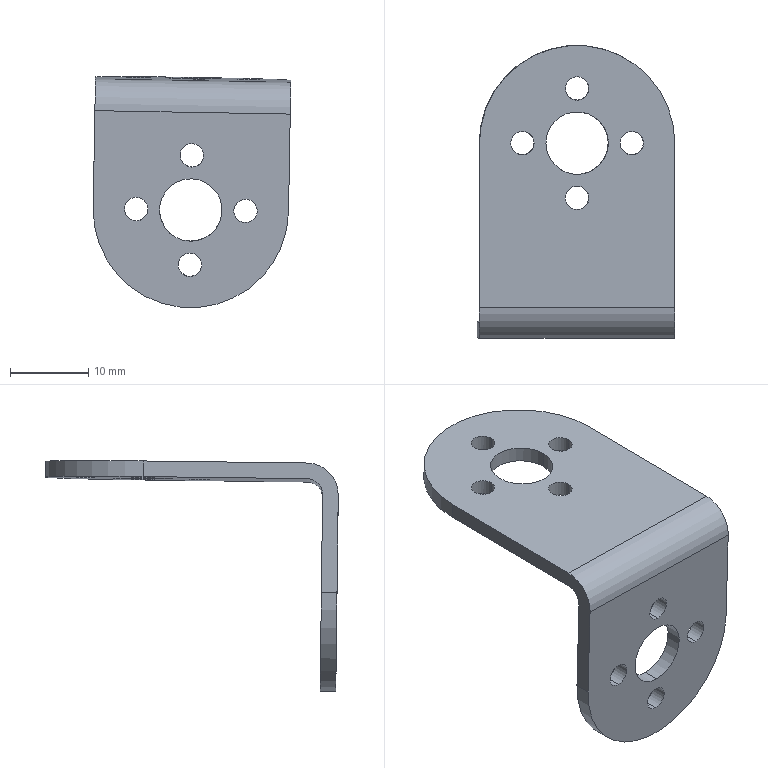Component | SolidWorks | L Shape Bracket-1 | 1 solid | 30 faces | box 25.29 x 37.47 x 29.58 mm | volume 2578 mm3 | cylinder 24 | plane 6 | commonest cylinder face diameters 3 x16 8 x5 25 x2 4 x1
STEP:
#1=COLOUR_RGB('',0.7922,0.8196,0.9333);
#2=FILL_AREA_STYLE_COLOUR('',#1);
#3=FILL_AREA_STYLE('',(#2));
#4=SURFACE_STYLE_FILL_AREA(#3);
#5=SURFACE_SIDE_STYLE('',(#4));
#6=SURFACE_STYLE_USAGE(.BOTH.,#5);
#7=PRESENTATION_STYLE_ASSIGNMENT((#6));
#8=CARTESIAN_POINT('',(1.258,4.504,1.069));
#9=VERTEX_POINT('',#8);
#10=CARTESIAN_POINT('',(1.261,4.659,1.228));
#11=VERTEX_POINT('',#10);
#12=CARTESIAN_POINT('',(1.258,4.661,1.071));
#13=DIRECTION('',(-0.9998,0.,0.01745));
#14=DIRECTION('',(0.01218,-0.716,0.698));
#15=AXIS2_PLACEMENT_3D('',#12,#13,#14);
#16=CIRCLE('',#15,0.1575);
#17=EDGE_CURVE('',#9,#11,#16,.T.);
#18=ORIENTED_EDGE('',*,*,#17,.T.);
#19=CARTESIAN_POINT('',(0.2769,4.659,1.246));
#20=VERTEX_POINT('',#19);
#21=CARTESIAN_POINT('',(0.5229,4.659,1.241));
#22=DIRECTION('',(-0.9998,0.,0.01745));
#23=VECTOR('',#22,39.37);
#24=LINE('',#21,#23);
#25=EDGE_CURVE('',#11,#20,#24,.T.);
#26=ORIENTED_EDGE('',*,*,#25,.T.);
#27=CARTESIAN_POINT('',(0.2741,4.504,1.086));
#28=VERTEX_POINT('',#27);
#29=CARTESIAN_POINT('',(0.2741,4.661,1.088));
#30=DIRECTION('',(0.9998,-0.,-0.01745));
#31=DIRECTION('',(0.01218,-0.716,0.698));
#32=AXIS2_PLACEMENT_3D('',#29,#30,#31);
#33=CIRCLE('',#32,0.1575);
#34=EDGE_CURVE('',#20,#28,#33,.T.);
#35=ORIENTED_EDGE('',*,*,#34,.T.);
#36=CARTESIAN_POINT('',(0.5201,4.504,1.082));
#37=DIRECTION('',(0.9998,-0.,-0.01745));
#38=VECTOR('',#37,39.37);
#39=LINE('',#36,#38);
#40=EDGE_CURVE('',#28,#9,#39,.T.);
#41=ORIENTED_EDGE('',*,*,#40,.T.);
#42=EDGE_LOOP('',(#18,#26,#35,#41));
#43=FACE_OUTER_BOUND('',#42,.T.);
#44=CARTESIAN_POINT('',(0.5202,4.661,1.084));
#45=DIRECTION('',(0.9998,-0.,-0.01745));
#46=DIRECTION('',(-0.01218,0.716,-0.698));
#47=AXIS2_PLACEMENT_3D('',#44,#45,#46);
#48=CYLINDRICAL_SURFACE('',#47,0.1575);
#49=ADVANCED_FACE('',(#43),#48,.T.);
#50=ORIENTED_EDGE('',*,*,#40,.F.);
#51=CARTESIAN_POINT('',(0.2655,4.51,0.5941));
#52=VERTEX_POINT('',#51);
#53=CARTESIAN_POINT('',(0.2755,4.503,1.165));
#54=DIRECTION('',(0.01745,-0.01259,0.9998));
#55=VECTOR('',#54,39.37);
#56=LINE('',#53,#55);
#57=EDGE_CURVE('',#52,#28,#56,.T.);
#58=ORIENTED_EDGE('',*,*,#57,.F.);
#59=CARTESIAN_POINT('',(1.25,4.51,0.5769));
#60=VERTEX_POINT('',#59);
#61=CARTESIAN_POINT('',(0.7576,4.51,0.5855));
#62=DIRECTION('',(-0.0002197,-0.9999,-0.01259));
#63=DIRECTION('',(-0.01745,0.01259,-0.9998));
#64=AXIS2_PLACEMENT_3D('',#61,#62,#63);
#65=CIRCLE('',#64,0.4921);
#66=EDGE_CURVE('',#52,#60,#65,.T.);
#67=ORIENTED_EDGE('',*,*,#66,.T.);
#68=CARTESIAN_POINT('',(1.26,4.503,1.148));
#69=DIRECTION('',(-0.01745,0.01259,-0.9998));
#70=VECTOR('',#69,39.37);
#71=LINE('',#68,#70);
#72=EDGE_CURVE('',#9,#60,#71,.T.);
#73=ORIENTED_EDGE('',*,*,#72,.F.);
#74=EDGE_LOOP('',(#50,#58,#67,#73));
#75=FACE_OUTER_BOUND('',#74,.T.);
#76=CARTESIAN_POINT('',(0.7634,4.506,0.9201));
#77=VERTEX_POINT('',#76);
#78=CARTESIAN_POINT('',(0.7613,4.507,0.802));
#79=VERTEX_POINT('',#78);
#80=CARTESIAN_POINT('',(0.7624,4.507,0.8611));
#81=DIRECTION('',(0.0002197,0.9999,0.01259));
#82=DIRECTION('',(-0.01745,0.01259,-0.9998));
#83=AXIS2_PLACEMENT_3D('',#80,#81,#82);
#84=CIRCLE('',#83,0.05906);
#85=EDGE_CURVE('',#77,#79,#84,.T.);
#86=ORIENTED_EDGE('',*,*,#85,.T.);
#87=CARTESIAN_POINT('',(0.7624,4.507,0.8611));
#88=DIRECTION('',(0.0002197,0.9999,0.01259));
#89=DIRECTION('',(-0.01745,0.01259,-0.9998));
#90=AXIS2_PLACEMENT_3D('',#87,#88,#89);
#91=CIRCLE('',#90,0.05906);
#92=EDGE_CURVE('',#79,#77,#91,.T.);
#93=ORIENTED_EDGE('',*,*,#92,.T.);
#94=EDGE_LOOP('',(#86,#93));
#95=FACE_BOUND('',#94,.T.);
#96=CARTESIAN_POINT('',(0.7603,4.508,0.743));
#97=VERTEX_POINT('',#96);
#98=CARTESIAN_POINT('',(0.7548,4.512,0.4281));
#99=VERTEX_POINT('',#98);
#100=CARTESIAN_POINT('',(0.7576,4.51,0.5855));
#101=DIRECTION('',(0.0002197,0.9999,0.01259));
#102=DIRECTION('',(-0.01745,0.01259,-0.9998));
#103=AXIS2_PLACEMENT_3D('',#100,#101,#102);
#104=CIRCLE('',#103,0.1575);
#105=EDGE_CURVE('',#97,#99,#104,.T.);
#106=ORIENTED_EDGE('',*,*,#105,.T.);
#107=CARTESIAN_POINT('',(0.7576,4.51,0.5855));
#108=DIRECTION('',(0.0002197,0.9999,0.01259));
#109=DIRECTION('',(-0.01745,0.01259,-0.9998));
#110=AXIS2_PLACEMENT_3D('',#107,#108,#109);
#111=CIRCLE('',#110,0.1575);
#112=EDGE_CURVE('',#99,#97,#111,.T.);
#113=ORIENTED_EDGE('',*,*,#112,.T.);
#114=EDGE_LOOP('',(#106,#113));
#115=FACE_BOUND('',#114,.T.);
#116=CARTESIAN_POINT('',(1.034,4.509,0.6398));
#117=VERTEX_POINT('',#116);
#118=CARTESIAN_POINT('',(1.032,4.511,0.5217));
#119=VERTEX_POINT('',#118);
#120=CARTESIAN_POINT('',(1.033,4.51,0.5807));
#121=DIRECTION('',(0.0002197,0.9999,0.01259));
#122=DIRECTION('',(-0.01745,0.01259,-0.9998));
#123=AXIS2_PLACEMENT_3D('',#120,#121,#122);
#124=CIRCLE('',#123,0.05906);
#125=EDGE_CURVE('',#117,#119,#124,.T.);
#126=ORIENTED_EDGE('',*,*,#125,.T.);
#127=CARTESIAN_POINT('',(1.033,4.51,0.5807));
#128=DIRECTION('',(0.0002197,0.9999,0.01259));
#129=DIRECTION('',(-0.01745,0.01259,-0.9998));
#130=AXIS2_PLACEMENT_3D('',#127,#128,#129);
#131=CIRCLE('',#130,0.05906);
#132=EDGE_CURVE('',#119,#117,#131,.T.);
#133=ORIENTED_EDGE('',*,*,#132,.T.);
#134=EDGE_LOOP('',(#126,#133));
#135=FACE_BOUND('',#134,.T.);
#136=CARTESIAN_POINT('',(0.4831,4.509,0.6494));
#137=VERTEX_POINT('',#136);
#138=CARTESIAN_POINT('',(0.481,4.511,0.5313));
#139=VERTEX_POINT('',#138);
#140=CARTESIAN_POINT('',(0.482,4.51,0.5903));
#141=DIRECTION('',(0.0002197,0.9999,0.01259));
#142=DIRECTION('',(-0.01745,0.01259,-0.9998));
#143=AXIS2_PLACEMENT_3D('',#140,#141,#142);
#144=CIRCLE('',#143,0.05906);
#145=EDGE_CURVE('',#137,#139,#144,.T.);
#146=ORIENTED_EDGE('',*,*,#145,.T.);
#147=CARTESIAN_POINT('',(0.482,4.51,0.5903));
#148=DIRECTION('',(0.0002197,0.9999,0.01259));
#149=DIRECTION('',(-0.01745,0.01259,-0.9998));
#150=AXIS2_PLACEMENT_3D('',#147,#148,#149);
#151=CIRCLE('',#150,0.05906);
#152=EDGE_CURVE('',#139,#137,#151,.T.);
#153=ORIENTED_EDGE('',*,*,#152,.T.);
#154=EDGE_LOOP('',(#146,#153));
#155=FACE_BOUND('',#154,.T.);
#156=CARTESIAN_POINT('',(0.7538,4.513,0.369));
#157=VERTEX_POINT('',#156);
#158=CARTESIAN_POINT('',(0.7517,4.514,0.251));
#159=VERTEX_POINT('',#158);
#160=CARTESIAN_POINT('',(0.7528,4.513,0.31));
#161=DIRECTION('',(0.0002197,0.9999,0.01259));
#162=DIRECTION('',(-0.01745,0.01259,-0.9998));
#163=AXIS2_PLACEMENT_3D('',#160,#161,#162);
#164=CIRCLE('',#163,0.05906);
#165=EDGE_CURVE('',#157,#159,#164,.T.);
#166=ORIENTED_EDGE('',*,*,#165,.T.);
#167=CARTESIAN_POINT('',(0.7528,4.513,0.31));
#168=DIRECTION('',(0.0002197,0.9999,0.01259));
#169=DIRECTION('',(-0.01745,0.01259,-0.9998));
#170=AXIS2_PLACEMENT_3D('',#167,#168,#169);
#171=CIRCLE('',#170,0.05906);
#172=EDGE_CURVE('',#159,#157,#171,.T.);
#173=ORIENTED_EDGE('',*,*,#172,.T.);
#174=EDGE_LOOP('',(#166,#173));
#175=FACE_BOUND('',#174,.T.);
#176=CARTESIAN_POINT('',(0.2755,4.503,1.165));
#177=DIRECTION('',(-0.0002197,-0.9999,-0.01259));
#178=DIRECTION('',(0.9998,-0.,-0.01745));
#179=AXIS2_PLACEMENT_3D('',#176,#177,#178);
#180=PLANE('',#179);
#181=ADVANCED_FACE('',(#75,#95,#115,#135,#155,#175),#180,.T.);
#182=CARTESIAN_POINT('',(0.7538,4.591,0.37));
#183=VERTEX_POINT('',#182);
#184=CARTESIAN_POINT('',(0.7538,4.591,0.37));
#185=DIRECTION('',(-0.0002197,-0.9999,-0.01259));
#186=VECTOR('',#185,39.37);
#187=LINE('',#184,#186);
#188=EDGE_CURVE('',#183,#157,#187,.T.);
#189=ORIENTED_EDGE('',*,*,#188,.T.);
#190=ORIENTED_EDGE('',*,*,#172,.F.);
#191=CARTESIAN_POINT('',(0.7517,4.593,0.252));
#192=VERTEX_POINT('',#191);
#193=CARTESIAN_POINT('',(0.7517,4.593,0.252));
#194=DIRECTION('',(-0.0002197,-0.9999,-0.01259));
#195=VECTOR('',#194,39.37);
#196=LINE('',#193,#195);
#197=EDGE_CURVE('',#192,#159,#196,.T.);
#198=ORIENTED_EDGE('',*,*,#197,.F.);
#199=CARTESIAN_POINT('',(0.7528,4.592,0.311));
#200=DIRECTION('',(-0.0002197,-0.9999,-0.01259));
#201=DIRECTION('',(-0.01745,0.01259,-0.9998));
#202=AXIS2_PLACEMENT_3D('',#199,#200,#201);
#203=CIRCLE('',#202,0.05906);
#204=EDGE_CURVE('',#183,#192,#203,.T.);
#205=ORIENTED_EDGE('',*,*,#204,.F.);
#206=EDGE_LOOP('',(#189,#190,#198,#205));
#207=FACE_OUTER_BOUND('',#206,.T.);
#208=CARTESIAN_POINT('',(0.7528,4.592,0.311));
#209=DIRECTION('',(-0.0002197,-0.9999,-0.01259));
#210=DIRECTION('',(0.9998,0.,-0.01745));
#211=AXIS2_PLACEMENT_3D('',#208,#209,#210);
#212=CYLINDRICAL_SURFACE('',#211,0.05906);
#213=ADVANCED_FACE('',(#207),#212,.F.);
#214=CARTESIAN_POINT('',(1.258,4.583,1.07));
#215=VERTEX_POINT('',#214);
#216=CARTESIAN_POINT('',(0.2741,4.583,1.087));
#217=VERTEX_POINT('',#216);
#218=CARTESIAN_POINT('',(0.5202,4.583,1.083));
#219=DIRECTION('',(-0.9998,0.,0.01745));
#220=VECTOR('',#219,39.37);
#221=LINE('',#218,#220);
#222=EDGE_CURVE('',#215,#217,#221,.T.);
#223=ORIENTED_EDGE('',*,*,#222,.F.);
#224=CARTESIAN_POINT('',(1.25,4.589,0.5779));
#225=VERTEX_POINT('',#224);
#226=CARTESIAN_POINT('',(1.26,4.582,1.149));
#227=DIRECTION('',(-0.01745,0.01259,-0.9998));
#228=VECTOR('',#227,39.37);
#229=LINE('',#226,#228);
#230=EDGE_CURVE('',#215,#225,#229,.T.);
#231=ORIENTED_EDGE('',*,*,#230,.T.);
#232=CARTESIAN_POINT('',(0.2655,4.589,0.5951));
#233=VERTEX_POINT('',#232);
#234=CARTESIAN_POINT('',(0.7576,4.589,0.5865));
#235=DIRECTION('',(0.0002197,0.9999,0.01259));
#236=DIRECTION('',(-0.01745,0.01259,-0.9998));
#237=AXIS2_PLACEMENT_3D('',#234,#235,#236);
#238=CIRCLE('',#237,0.4921);
#239=EDGE_CURVE('',#225,#233,#238,.T.);
#240=ORIENTED_EDGE('',*,*,#239,.T.);
#241=CARTESIAN_POINT('',(0.2755,4.582,1.166));
#242=DIRECTION('',(-0.01745,0.01259,-0.9998));
#243=VECTOR('',#242,39.37);
#244=LINE('',#241,#243);
#245=EDGE_CURVE('',#217,#233,#244,.T.);
#246=ORIENTED_EDGE('',*,*,#245,.F.);
#247=EDGE_LOOP('',(#223,#231,#240,#246));
#248=FACE_OUTER_BOUND('',#247,.T.);
#249=ORIENTED_EDGE('',*,*,#204,.T.);
#250=CARTESIAN_POINT('',(0.7528,4.592,0.311));
#251=DIRECTION('',(-0.0002197,-0.9999,-0.01259));
#252=DIRECTION('',(-0.01745,0.01259,-0.9998));
#253=AXIS2_PLACEMENT_3D('',#250,#251,#252);
#254=CIRCLE('',#253,0.05906);
#255=EDGE_CURVE('',#192,#183,#254,.T.);
#256=ORIENTED_EDGE('',*,*,#255,.T.);
#257=EDGE_LOOP('',(#249,#256));
#258=FACE_BOUND('',#257,.T.);
#259=CARTESIAN_POINT('',(0.4831,4.588,0.6504));
#260=VERTEX_POINT('',#259);
#261=CARTESIAN_POINT('',(0.481,4.589,0.5323));
#262=VERTEX_POINT('',#261);
#263=CARTESIAN_POINT('',(0.482,4.589,0.5913));
#264=DIRECTION('',(-0.0002197,-0.9999,-0.01259));
#265=DIRECTION('',(-0.01745,0.01259,-0.9998));
#266=AXIS2_PLACEMENT_3D('',#263,#264,#265);
#267=CIRCLE('',#266,0.05906);
#268=EDGE_CURVE('',#260,#262,#267,.T.);
#269=ORIENTED_EDGE('',*,*,#268,.T.);
#270=CARTESIAN_POINT('',(0.482,4.589,0.5913));
#271=DIRECTION('',(-0.0002197,-0.9999,-0.01259));
#272=DIRECTION('',(-0.01745,0.01259,-0.9998));
#273=AXIS2_PLACEMENT_3D('',#270,#271,#272);
#274=CIRCLE('',#273,0.05906);
#275=EDGE_CURVE('',#262,#260,#274,.T.);
#276=ORIENTED_EDGE('',*,*,#275,.T.);
#277=EDGE_LOOP('',(#269,#276));
#278=FACE_BOUND('',#277,.T.);
#279=CARTESIAN_POINT('',(1.034,4.588,0.6407));
#280=VERTEX_POINT('',#279);
#281=CARTESIAN_POINT('',(1.032,4.589,0.5227));
#282=VERTEX_POINT('',#281);
#283=CARTESIAN_POINT('',(1.033,4.589,0.5817));
#284=DIRECTION('',(-0.0002197,-0.9999,-0.01259));
#285=DIRECTION('',(-0.01745,0.01259,-0.9998));
#286=AXIS2_PLACEMENT_3D('',#283,#284,#285);
#287=CIRCLE('',#286,0.05906);
#288=EDGE_CURVE('',#280,#282,#287,.T.);
#289=ORIENTED_EDGE('',*,*,#288,.T.);
#290=CARTESIAN_POINT('',(1.033,4.589,0.5817));
#291=DIRECTION('',(-0.0002197,-0.9999,-0.01259));
#292=DIRECTION('',(-0.01745,0.01259,-0.9998));
#293=AXIS2_PLACEMENT_3D('',#290,#291,#292);
#294=CIRCLE('',#293,0.05906);
#295=EDGE_CURVE('',#282,#280,#294,.T.);
#296=ORIENTED_EDGE('',*,*,#295,.T.);
#297=EDGE_LOOP('',(#289,#296));
#298=FACE_BOUND('',#297,.T.);
#299=CARTESIAN_POINT('',(0.7603,4.587,0.744));
#300=VERTEX_POINT('',#299);
#301=CARTESIAN_POINT('',(0.7548,4.591,0.4291));
#302=VERTEX_POINT('',#301);
#303=CARTESIAN_POINT('',(0.7576,4.589,0.5865));
#304=DIRECTION('',(-0.0002197,-0.9999,-0.01259));
#305=DIRECTION('',(-0.01745,0.01259,-0.9998));
#306=AXIS2_PLACEMENT_3D('',#303,#304,#305);
#307=CIRCLE('',#306,0.1575);
#308=EDGE_CURVE('',#300,#302,#307,.T.);
#309=ORIENTED_EDGE('',*,*,#308,.T.);
#310=CARTESIAN_POINT('',(0.7576,4.589,0.5865));
#311=DIRECTION('',(-0.0002197,-0.9999,-0.01259));
#312=DIRECTION('',(-0.01745,0.01259,-0.9998));
#313=AXIS2_PLACEMENT_3D('',#310,#311,#312);
#314=CIRCLE('',#313,0.1575);
#315=EDGE_CURVE('',#302,#300,#314,.T.);
#316=ORIENTED_EDGE('',*,*,#315,.T.);
#317=EDGE_LOOP('',(#309,#316));
#318=FACE_BOUND('',#317,.T.);
#319=CARTESIAN_POINT('',(0.7634,4.585,0.9211));
#320=VERTEX_POINT('',#319);
#321=CARTESIAN_POINT('',(0.7614,4.586,0.803));
#322=VERTEX_POINT('',#321);
#323=CARTESIAN_POINT('',(0.7624,4.585,0.862));
#324=DIRECTION('',(-0.0002197,-0.9999,-0.01259));
#325=DIRECTION('',(-0.01745,0.01259,-0.9998));
#326=AXIS2_PLACEMENT_3D('',#323,#324,#325);
#327=CIRCLE('',#326,0.05906);
#328=EDGE_CURVE('',#320,#322,#327,.T.);
#329=ORIENTED_EDGE('',*,*,#328,.T.);
#330=CARTESIAN_POINT('',(0.7624,4.585,0.862));
#331=DIRECTION('',(-0.0002197,-0.9999,-0.01259));
#332=DIRECTION('',(-0.01745,0.01259,-0.9998));
#333=AXIS2_PLACEMENT_3D('',#330,#331,#332);
#334=CIRCLE('',#333,0.05906);
#335=EDGE_CURVE('',#322,#320,#334,.T.);
#336=ORIENTED_EDGE('',*,*,#335,.T.);
#337=EDGE_LOOP('',(#329,#336));
#338=FACE_BOUND('',#337,.T.);
#339=CARTESIAN_POINT('',(0.2755,4.582,1.166));
#340=DIRECTION('',(0.0002197,0.9999,0.01259));
#341=DIRECTION('',(0.9998,-0.,-0.01745));
#342=AXIS2_PLACEMENT_3D('',#339,#340,#341);
#343=PLANE('',#342);
#344=ADVANCED_FACE('',(#248,#258,#278,#298,#318,#338),#343,.T.);
#345=CARTESIAN_POINT('',(0.7634,4.585,0.9211));
#346=DIRECTION('',(-0.0002197,-0.9999,-0.01259));
#347=VECTOR('',#346,39.37);
#348=LINE('',#345,#347);
#349=EDGE_CURVE('',#320,#77,#348,.T.);
#350=ORIENTED_EDGE('',*,*,#349,.F.);
#351=ORIENTED_EDGE('',*,*,#335,.F.);
#352=CARTESIAN_POINT('',(0.7614,4.586,0.803));
#353=DIRECTION('',(-0.0002197,-0.9999,-0.01259));
#354=VECTOR('',#353,39.37);
#355=LINE('',#352,#354);
#356=EDGE_CURVE('',#322,#79,#355,.T.);
#357=ORIENTED_EDGE('',*,*,#356,.T.);
#358=ORIENTED_EDGE('',*,*,#85,.F.);
#359=EDGE_LOOP('',(#350,#351,#357,#358));
#360=FACE_OUTER_BOUND('',#359,.T.);
#361=CARTESIAN_POINT('',(0.7624,4.585,0.862));
#362=DIRECTION('',(-0.0002197,-0.9999,-0.01259));
#363=DIRECTION('',(-0.9998,0.,0.01745));
#364=AXIS2_PLACEMENT_3D('',#361,#362,#363);
#365=CYLINDRICAL_SURFACE('',#364,0.05906);
#366=ADVANCED_FACE('',(#360),#365,.F.);
#367=ORIENTED_EDGE('',*,*,#349,.T.);
#368=ORIENTED_EDGE('',*,*,#92,.F.);
#369=ORIENTED_EDGE('',*,*,#356,.F.);
#370=ORIENTED_EDGE('',*,*,#328,.F.);
#371=EDGE_LOOP('',(#367,#368,#369,#370));
#372=FACE_OUTER_BOUND('',#371,.T.);
#373=CARTESIAN_POINT('',(0.7624,4.585,0.862));
#374=DIRECTION('',(-0.0002197,-0.9999,-0.01259));
#375=DIRECTION('',(0.9998,0.,-0.01745));
#376=AXIS2_PLACEMENT_3D('',#373,#374,#375);
#377=CYLINDRICAL_SURFACE('',#376,0.05906);
#378=ADVANCED_FACE('',(#372),#377,.F.);
#379=CARTESIAN_POINT('',(0.7603,4.587,0.744));
#380=DIRECTION('',(-0.0002197,-0.9999,-0.01259));
#381=VECTOR('',#380,39.37);
#382=LINE('',#379,#381);
#383=EDGE_CURVE('',#300,#97,#382,.T.);
#384=ORIENTED_EDGE('',*,*,#383,.F.);
#385=ORIENTED_EDGE('',*,*,#315,.F.);
#386=CARTESIAN_POINT('',(0.7548,4.591,0.4291));
#387=DIRECTION('',(-0.0002197,-0.9999,-0.01259));
#388=VECTOR('',#387,39.37);
#389=LINE('',#386,#388);
#390=EDGE_CURVE('',#302,#99,#389,.T.);
#391=ORIENTED_EDGE('',*,*,#390,.T.);
#392=ORIENTED_EDGE('',*,*,#105,.F.);
#393=EDGE_LOOP('',(#384,#385,#391,#392));
#394=FACE_OUTER_BOUND('',#393,.T.);
#395=CARTESIAN_POINT('',(0.7576,4.589,0.5865));
#396=DIRECTION('',(-0.0002197,-0.9999,-0.01259));
#397=DIRECTION('',(-0.9998,0.,0.01745));
#398=AXIS2_PLACEMENT_3D('',#395,#396,#397);
#399=CYLINDRICAL_SURFACE('',#398,0.1575);
#400=ADVANCED_FACE('',(#394),#399,.F.);
#401=ORIENTED_EDGE('',*,*,#383,.T.);
#402=ORIENTED_EDGE('',*,*,#112,.F.);
#403=ORIENTED_EDGE('',*,*,#390,.F.);
#404=ORIENTED_EDGE('',*,*,#308,.F.);
#405=EDGE_LOOP('',(#401,#402,#403,#404));
#406=FACE_OUTER_BOUND('',#405,.T.);
#407=CARTESIAN_POINT('',(0.7576,4.589,0.5865));
#408=DIRECTION('',(-0.0002197,-0.9999,-0.01259));
#409=DIRECTION('',(0.9998,-0.,-0.01745));
#410=AXIS2_PLACEMENT_3D('',#407,#408,#409);
#411=CYLINDRICAL_SURFACE('',#410,0.1575);
#412=ADVANCED_FACE('',(#406),#411,.F.);
#413=CARTESIAN_POINT('',(1.034,4.588,0.6407));
#414=DIRECTION('',(-0.0002197,-0.9999,-0.01259));
#415=VECTOR('',#414,39.37);
#416=LINE('',#413,#415);
#417=EDGE_CURVE('',#280,#117,#416,.T.);
#418=ORIENTED_EDGE('',*,*,#417,.F.);
#419=ORIENTED_EDGE('',*,*,#295,.F.);
#420=CARTESIAN_POINT('',(1.032,4.589,0.5227));
#421=DIRECTION('',(-0.0002197,-0.9999,-0.01259));
#422=VECTOR('',#421,39.37);
#423=LINE('',#420,#422);
#424=EDGE_CURVE('',#282,#119,#423,.T.);
#425=ORIENTED_EDGE('',*,*,#424,.T.);
#426=ORIENTED_EDGE('',*,*,#125,.F.);
#427=EDGE_LOOP('',(#418,#419,#425,#426));
#428=FACE_OUTER_BOUND('',#427,.T.);
#429=CARTESIAN_POINT('',(1.033,4.589,0.5817));
#430=DIRECTION('',(-0.0002197,-0.9999,-0.01259));
#431=DIRECTION('',(-0.9998,0.,0.01745));
#432=AXIS2_PLACEMENT_3D('',#429,#430,#431);
#433=CYLINDRICAL_SURFACE('',#432,0.05906);
#434=ADVANCED_FACE('',(#428),#433,.F.);
#435=ORIENTED_EDGE('',*,*,#417,.T.);
#436=ORIENTED_EDGE('',*,*,#132,.F.);
#437=ORIENTED_EDGE('',*,*,#424,.F.);
#438=ORIENTED_EDGE('',*,*,#288,.F.);
#439=EDGE_LOOP('',(#435,#436,#437,#438));
#440=FACE_OUTER_BOUND('',#439,.T.);
#441=CARTESIAN_POINT('',(1.033,4.589,0.5817));
#442=DIRECTION('',(-0.0002197,-0.9999,-0.01259));
#443=DIRECTION('',(0.9998,0.,-0.01745));
#444=AXIS2_PLACEMENT_3D('',#441,#442,#443);
#445=CYLINDRICAL_SURFACE('',#444,0.05906);
#446=ADVANCED_FACE('',(#440),#445,.F.);
#447=CARTESIAN_POINT('',(0.4831,4.588,0.6504));
#448=DIRECTION('',(-0.0002197,-0.9999,-0.01259));
#449=VECTOR('',#448,39.37);
#450=LINE('',#447,#449);
#451=EDGE_CURVE('',#260,#137,#450,.T.);
#452=ORIENTED_EDGE('',*,*,#451,.F.);
#453=ORIENTED_EDGE('',*,*,#275,.F.);
#454=CARTESIAN_POINT('',(0.481,4.589,0.5323));
#455=DIRECTION('',(-0.0002197,-0.9999,-0.01259));
#456=VECTOR('',#455,39.37);
#457=LINE('',#454,#456);
#458=EDGE_CURVE('',#262,#139,#457,.T.);
#459=ORIENTED_EDGE('',*,*,#458,.T.);
#460=ORIENTED_EDGE('',*,*,#145,.F.);
#461=EDGE_LOOP('',(#452,#453,#459,#460));
#462=FACE_OUTER_BOUND('',#461,.T.);
#463=CARTESIAN_POINT('',(0.482,4.589,0.5913));
#464=DIRECTION('',(-0.0002197,-0.9999,-0.01259));
#465=DIRECTION('',(-0.9998,0.,0.01745));
#466=AXIS2_PLACEMENT_3D('',#463,#464,#465);
#467=CYLINDRICAL_SURFACE('',#466,0.05906);
#468=ADVANCED_FACE('',(#462),#467,.F.);
#469=ORIENTED_EDGE('',*,*,#451,.T.);
#470=ORIENTED_EDGE('',*,*,#152,.F.);
#471=ORIENTED_EDGE('',*,*,#458,.F.);
#472=ORIENTED_EDGE('',*,*,#268,.F.);
#473=EDGE_LOOP('',(#469,#470,#471,#472));
#474=FACE_OUTER_BOUND('',#473,.T.);
#475=CARTESIAN_POINT('',(0.482,4.589,0.5913));
#476=DIRECTION('',(-0.0002197,-0.9999,-0.01259));
#477=DIRECTION('',(0.9998,0.,-0.01745));
#478=AXIS2_PLACEMENT_3D('',#475,#476,#477);
#479=CYLINDRICAL_SURFACE('',#478,0.05906);
#480=ADVANCED_FACE('',(#474),#479,.F.);
#481=ORIENTED_EDGE('',*,*,#188,.F.);
#482=ORIENTED_EDGE('',*,*,#255,.F.);
#483=ORIENTED_EDGE('',*,*,#197,.T.);
#484=ORIENTED_EDGE('',*,*,#165,.F.);
#485=EDGE_LOOP('',(#481,#482,#483,#484));
#486=FACE_OUTER_BOUND('',#485,.T.);
#487=CARTESIAN_POINT('',(0.7528,4.592,0.311));
#488=DIRECTION('',(-0.0002197,-0.9999,-0.01259));
#489=DIRECTION('',(-0.9998,0.,0.01745));
#490=AXIS2_PLACEMENT_3D('',#487,#488,#489);
#491=CYLINDRICAL_SURFACE('',#490,0.05906);
#492=ADVANCED_FACE('',(#486),#491,.F.);
#493=ORIENTED_EDGE('',*,*,#34,.F.);
#494=CARTESIAN_POINT('',(0.2771,5.486,1.256));
#495=VERTEX_POINT('',#494);
#496=CARTESIAN_POINT('',(0.2769,4.502,1.244));
#497=DIRECTION('',(-0.0002197,-0.9999,-0.01259));
#498=VECTOR('',#497,39.37);
#499=LINE('',#496,#498);
#500=EDGE_CURVE('',#495,#20,#499,.T.);
#501=ORIENTED_EDGE('',*,*,#500,.F.);
#502=CARTESIAN_POINT('',(0.2757,5.487,1.177));
#503=VERTEX_POINT('',#502);
#504=CARTESIAN_POINT('',(0.2757,5.487,1.177));
#505=DIRECTION('',(0.01745,-0.01259,0.9998));
#506=VECTOR('',#505,39.37);
#507=LINE('',#504,#506);
#508=EDGE_CURVE('',#503,#495,#507,.T.);
#509=ORIENTED_EDGE('',*,*,#508,.F.);
#510=CARTESIAN_POINT('',(0.2755,4.66,1.167));
#511=VERTEX_POINT('',#510);
#512=CARTESIAN_POINT('',(0.2755,4.503,1.165));
#513=DIRECTION('',(0.0002197,0.9999,0.01259));
#514=VECTOR('',#513,39.37);
#515=LINE('',#512,#514);
#516=EDGE_CURVE('',#511,#503,#515,.T.);
#517=ORIENTED_EDGE('',*,*,#516,.F.);
#518=CARTESIAN_POINT('',(0.2741,4.661,1.088));
#519=DIRECTION('',(-0.9998,0.,0.01745));
#520=DIRECTION('',(0.01218,-0.716,0.698));
#521=AXIS2_PLACEMENT_3D('',#518,#519,#520);
#522=CIRCLE('',#521,0.07874);
#523=EDGE_CURVE('',#217,#511,#522,.T.);
#524=ORIENTED_EDGE('',*,*,#523,.F.);
#525=ORIENTED_EDGE('',*,*,#245,.T.);
#526=CARTESIAN_POINT('',(0.2655,4.589,0.5951));
#527=DIRECTION('',(0.0002197,0.9999,0.01259));
#528=VECTOR('',#527,39.37);
#529=LINE('',#526,#528);
#530=EDGE_CURVE('',#52,#233,#529,.T.);
#531=ORIENTED_EDGE('',*,*,#530,.F.);
#532=ORIENTED_EDGE('',*,*,#57,.T.);
#533=EDGE_LOOP('',(#493,#501,#509,#517,#524,#525,#531,#532));
#534=FACE_OUTER_BOUND('',#533,.T.);
#535=CARTESIAN_POINT('',(0.2757,5.487,1.177));
#536=DIRECTION('',(-0.9998,0.,0.01745));
#537=DIRECTION('',(-0.0002197,-0.9999,-0.01259));
#538=AXIS2_PLACEMENT_3D('',#535,#536,#537);
#539=PLANE('',#538);
#540=ADVANCED_FACE('',(#534),#539,.T.);
#541=ORIENTED_EDGE('',*,*,#239,.F.);
#542=CARTESIAN_POINT('',(1.25,4.589,0.5779));
#543=DIRECTION('',(0.0002197,0.9999,0.01259));
#544=VECTOR('',#543,39.37);
#545=LINE('',#542,#544);
#546=EDGE_CURVE('',#60,#225,#545,.T.);
#547=ORIENTED_EDGE('',*,*,#546,.F.);
#548=ORIENTED_EDGE('',*,*,#66,.F.);
#549=ORIENTED_EDGE('',*,*,#530,.T.);
#550=EDGE_LOOP('',(#541,#547,#548,#549));
#551=FACE_OUTER_BOUND('',#550,.T.);
#552=CARTESIAN_POINT('',(0.7576,4.589,0.5865));
#553=DIRECTION('',(-0.0002197,-0.9999,-0.01259));
#554=DIRECTION('',(0.01745,-0.01259,0.9998));
#555=AXIS2_PLACEMENT_3D('',#552,#553,#554);
#556=CYLINDRICAL_SURFACE('',#555,0.4921);
#557=ADVANCED_FACE('',(#551),#556,.T.);
#558=ORIENTED_EDGE('',*,*,#17,.F.);
#559=ORIENTED_EDGE('',*,*,#72,.T.);
#560=ORIENTED_EDGE('',*,*,#546,.T.);
#561=ORIENTED_EDGE('',*,*,#230,.F.);
#562=CARTESIAN_POINT('',(1.26,4.66,1.15));
#563=VERTEX_POINT('',#562);
#564=CARTESIAN_POINT('',(1.258,4.661,1.071));
#565=DIRECTION('',(0.9998,-0.,-0.01745));
#566=DIRECTION('',(0.01218,-0.716,0.698));
#567=AXIS2_PLACEMENT_3D('',#564,#565,#566);
#568=CIRCLE('',#567,0.07874);
#569=EDGE_CURVE('',#563,#215,#568,.T.);
#570=ORIENTED_EDGE('',*,*,#569,.F.);
#571=CARTESIAN_POINT('',(1.26,5.487,1.16));
#572=VERTEX_POINT('',#571);
#573=CARTESIAN_POINT('',(1.26,5.979,1.166));
#574=DIRECTION('',(-0.0002197,-0.9999,-0.01259));
#575=VECTOR('',#574,39.37);
#576=LINE('',#573,#575);
#577=EDGE_CURVE('',#572,#563,#576,.T.);
#578=ORIENTED_EDGE('',*,*,#577,.F.);
#579=CARTESIAN_POINT('',(1.261,5.486,1.239));
#580=VERTEX_POINT('',#579);
#581=CARTESIAN_POINT('',(1.26,5.487,1.16));
#582=DIRECTION('',(0.01745,-0.01259,0.9998));
#583=VECTOR('',#582,39.37);
#584=LINE('',#581,#583);
#585=EDGE_CURVE('',#572,#580,#584,.T.);
#586=ORIENTED_EDGE('',*,*,#585,.T.);
#587=CARTESIAN_POINT('',(1.261,5.978,1.245));
#588=DIRECTION('',(0.0002197,0.9999,0.01259));
#589=VECTOR('',#588,39.37);
#590=LINE('',#587,#589);
#591=EDGE_CURVE('',#11,#580,#590,.T.);
#592=ORIENTED_EDGE('',*,*,#591,.F.);
#593=EDGE_LOOP('',(#558,#559,#560,#561,#570,#578,#586,#592));
#594=FACE_OUTER_BOUND('',#593,.T.);
#595=CARTESIAN_POINT('',(1.26,4.503,1.148));
#596=DIRECTION('',(0.9998,-0.,-0.01745));
#597=DIRECTION('',(0.0002197,0.9999,0.01259));
#598=AXIS2_PLACEMENT_3D('',#595,#596,#597);
#599=PLANE('',#598);
#600=ADVANCED_FACE('',(#594),#599,.T.);
#601=ORIENTED_EDGE('',*,*,#25,.F.);
#602=ORIENTED_EDGE('',*,*,#591,.T.);
#603=CARTESIAN_POINT('',(0.7691,5.486,1.247));
#604=DIRECTION('',(0.01745,-0.01259,0.9998));
#605=DIRECTION('',(0.9998,-0.,-0.01745));
#606=AXIS2_PLACEMENT_3D('',#603,#604,#605);
#607=CIRCLE('',#606,0.4921);
#608=EDGE_CURVE('',#580,#495,#607,.T.);
#609=ORIENTED_EDGE('',*,*,#608,.T.);
#610=ORIENTED_EDGE('',*,*,#500,.T.);
#611=EDGE_LOOP('',(#601,#602,#609,#610));
#612=FACE_OUTER_BOUND('',#611,.T.);
#613=CARTESIAN_POINT('',(0.6117,5.486,1.25));
#614=VERTEX_POINT('',#613);
#615=CARTESIAN_POINT('',(0.9266,5.486,1.245));
#616=VERTEX_POINT('',#615);
#617=CARTESIAN_POINT('',(0.7691,5.486,1.247));
#618=DIRECTION('',(-0.01745,0.01259,-0.9998));
#619=DIRECTION('',(0.9998,0.,-0.01745));
#620=AXIS2_PLACEMENT_3D('',#617,#618,#619);
#621=CIRCLE('',#620,0.1575);
#622=EDGE_CURVE('',#614,#616,#621,.T.);
#623=ORIENTED_EDGE('',*,*,#622,.T.);
#624=CARTESIAN_POINT('',(0.7691,5.486,1.247));
#625=DIRECTION('',(-0.01745,0.01259,-0.9998));
#626=DIRECTION('',(0.9998,0.,-0.01745));
#627=AXIS2_PLACEMENT_3D('',#624,#625,#626);
#628=CIRCLE('',#627,0.1575);
#629=EDGE_CURVE('',#616,#614,#628,.T.);
#630=ORIENTED_EDGE('',*,*,#629,.T.);
#631=EDGE_LOOP('',(#623,#630));
#632=FACE_BOUND('',#631,.T.);
#633=CARTESIAN_POINT('',(0.71,5.21,1.245));
#634=VERTEX_POINT('',#633);
#635=CARTESIAN_POINT('',(0.8281,5.21,1.243));
#636=VERTEX_POINT('',#635);
#637=CARTESIAN_POINT('',(0.7691,5.21,1.244));
#638=DIRECTION('',(-0.01745,0.01259,-0.9998));
#639=DIRECTION('',(0.9998,0.,-0.01745));
#640=AXIS2_PLACEMENT_3D('',#637,#638,#639);
#641=CIRCLE('',#640,0.05906);
#642=EDGE_CURVE('',#634,#636,#641,.T.);
#643=ORIENTED_EDGE('',*,*,#642,.T.);
#644=CARTESIAN_POINT('',(0.7691,5.21,1.244));
#645=DIRECTION('',(-0.01745,0.01259,-0.9998));
#646=DIRECTION('',(0.9998,0.,-0.01745));
#647=AXIS2_PLACEMENT_3D('',#644,#645,#646);
#648=CIRCLE('',#647,0.05906);
#649=EDGE_CURVE('',#636,#634,#648,.T.);
#650=ORIENTED_EDGE('',*,*,#649,.T.);
#651=EDGE_LOOP('',(#643,#650));
#652=FACE_BOUND('',#651,.T.);
#653=CARTESIAN_POINT('',(0.7101,5.762,1.252));
#654=VERTEX_POINT('',#653);
#655=CARTESIAN_POINT('',(0.8282,5.762,1.25));
#656=VERTEX_POINT('',#655);
#657=CARTESIAN_POINT('',(0.7692,5.762,1.251));
#658=DIRECTION('',(-0.01745,0.01259,-0.9998));
#659=DIRECTION('',(0.9998,0.,-0.01745));
#660=AXIS2_PLACEMENT_3D('',#657,#658,#659);
#661=CIRCLE('',#660,0.05906);
#662=EDGE_CURVE('',#654,#656,#661,.T.);
#663=ORIENTED_EDGE('',*,*,#662,.T.);
#664=CARTESIAN_POINT('',(0.7692,5.762,1.251));
#665=DIRECTION('',(-0.01745,0.01259,-0.9998));
#666=DIRECTION('',(0.9998,0.,-0.01745));
#667=AXIS2_PLACEMENT_3D('',#664,#665,#666);
#668=CIRCLE('',#667,0.05906);
#669=EDGE_CURVE('',#656,#654,#668,.T.);
#670=ORIENTED_EDGE('',*,*,#669,.T.);
#671=EDGE_LOOP('',(#663,#670));
#672=FACE_BOUND('',#671,.T.);
#673=CARTESIAN_POINT('',(0.9856,5.486,1.244));
#674=VERTEX_POINT('',#673);
#675=CARTESIAN_POINT('',(1.104,5.486,1.242));
#676=VERTEX_POINT('',#675);
#677=CARTESIAN_POINT('',(1.045,5.486,1.243));
#678=DIRECTION('',(-0.01745,0.01259,-0.9998));
#679=DIRECTION('',(0.9998,0.,-0.01745));
#680=AXIS2_PLACEMENT_3D('',#677,#678,#679);
#681=CIRCLE('',#680,0.05906);
#682=EDGE_CURVE('',#674,#676,#681,.T.);
#683=ORIENTED_EDGE('',*,*,#682,.T.);
#684=CARTESIAN_POINT('',(1.045,5.486,1.243));
#685=DIRECTION('',(-0.01745,0.01259,-0.9998));
#686=DIRECTION('',(0.9998,0.,-0.01745));
#687=AXIS2_PLACEMENT_3D('',#684,#685,#686);
#688=CIRCLE('',#687,0.05906);
#689=EDGE_CURVE('',#676,#674,#688,.T.);
#690=ORIENTED_EDGE('',*,*,#689,.T.);
#691=EDGE_LOOP('',(#683,#690));
#692=FACE_BOUND('',#691,.T.);
#693=CARTESIAN_POINT('',(0.4345,5.486,1.253));
#694=VERTEX_POINT('',#693);
#695=CARTESIAN_POINT('',(0.5526,5.486,1.251));
#696=VERTEX_POINT('',#695);
#697=CARTESIAN_POINT('',(0.4936,5.486,1.252));
#698=DIRECTION('',(-0.01745,0.01259,-0.9998));
#699=DIRECTION('',(0.9998,0.,-0.01745));
#700=AXIS2_PLACEMENT_3D('',#697,#698,#699);
#701=CIRCLE('',#700,0.05906);
#702=EDGE_CURVE('',#694,#696,#701,.T.);
#703=ORIENTED_EDGE('',*,*,#702,.T.);
#704=CARTESIAN_POINT('',(0.4936,5.486,1.252));
#705=DIRECTION('',(-0.01745,0.01259,-0.9998));
#706=DIRECTION('',(0.9998,0.,-0.01745));
#707=AXIS2_PLACEMENT_3D('',#704,#705,#706);
#708=CIRCLE('',#707,0.05906);
#709=EDGE_CURVE('',#696,#694,#708,.T.);
#710=ORIENTED_EDGE('',*,*,#709,.T.);
#711=EDGE_LOOP('',(#703,#710));
#712=FACE_BOUND('',#711,.T.);
#713=CARTESIAN_POINT('',(0.7691,5.24,1.244));
#714=DIRECTION('',(0.01745,-0.01259,0.9998));
#715=DIRECTION('',(0.9998,-0.,-0.01745));
#716=AXIS2_PLACEMENT_3D('',#713,#714,#715);
#717=PLANE('',#716);
#718=ADVANCED_FACE('',(#612,#632,#652,#672,#692,#712),#717,.T.);
#719=CARTESIAN_POINT('',(0.4332,5.487,1.174));
#720=VERTEX_POINT('',#719);
#721=CARTESIAN_POINT('',(0.4332,5.487,1.174));
#722=DIRECTION('',(0.01745,-0.01259,0.9998));
#723=VECTOR('',#722,39.37);
#724=LINE('',#721,#723);
#725=EDGE_CURVE('',#720,#694,#724,.T.);
#726=ORIENTED_EDGE('',*,*,#725,.T.);
#727=ORIENTED_EDGE('',*,*,#709,.F.);
#728=CARTESIAN_POINT('',(0.5512,5.487,1.172));
#729=VERTEX_POINT('',#728);
#730=CARTESIAN_POINT('',(0.5512,5.487,1.172));
#731=DIRECTION('',(0.01745,-0.01259,0.9998));
#732=VECTOR('',#731,39.37);
#733=LINE('',#730,#732);
#734=EDGE_CURVE('',#729,#696,#733,.T.);
#735=ORIENTED_EDGE('',*,*,#734,.F.);
#736=CARTESIAN_POINT('',(0.4922,5.487,1.173));
#737=DIRECTION('',(-0.01745,0.01259,-0.9998));
#738=DIRECTION('',(0.9998,0.,-0.01745));
#739=AXIS2_PLACEMENT_3D('',#736,#737,#738);
#740=CIRCLE('',#739,0.05906);
#741=EDGE_CURVE('',#729,#720,#740,.T.);
#742=ORIENTED_EDGE('',*,*,#741,.T.);
#743=EDGE_LOOP('',(#726,#727,#735,#742));
#744=FACE_OUTER_BOUND('',#743,.T.);
#745=CARTESIAN_POINT('',(0.4922,5.487,1.173));
#746=DIRECTION('',(0.01745,-0.01259,0.9998));
#747=DIRECTION('',(0.0002197,0.9999,0.01259));
#748=AXIS2_PLACEMENT_3D('',#745,#746,#747);
#749=CYLINDRICAL_SURFACE('',#748,0.05906);
#750=ADVANCED_FACE('',(#744),#749,.F.);
#751=CARTESIAN_POINT('',(0.5215,4.66,1.163));
#752=DIRECTION('',(0.9998,-0.,-0.01745));
#753=VECTOR('',#752,39.37);
#754=LINE('',#751,#753);
#755=EDGE_CURVE('',#511,#563,#754,.T.);
#756=ORIENTED_EDGE('',*,*,#755,.F.);
#757=ORIENTED_EDGE('',*,*,#516,.T.);
#758=CARTESIAN_POINT('',(0.7677,5.487,1.169));
#759=DIRECTION('',(0.01745,-0.01259,0.9998));
#760=DIRECTION('',(0.9998,-0.,-0.01745));
#761=AXIS2_PLACEMENT_3D('',#758,#759,#760);
#762=CIRCLE('',#761,0.4921);
#763=EDGE_CURVE('',#572,#503,#762,.T.);
#764=ORIENTED_EDGE('',*,*,#763,.F.);
#765=ORIENTED_EDGE('',*,*,#577,.T.);
#766=EDGE_LOOP('',(#756,#757,#764,#765));
#767=FACE_OUTER_BOUND('',#766,.T.);
#768=ORIENTED_EDGE('',*,*,#741,.F.);
#769=CARTESIAN_POINT('',(0.4922,5.487,1.173));
#770=DIRECTION('',(-0.01745,0.01259,-0.9998));
#771=DIRECTION('',(0.9998,0.,-0.01745));
#772=AXIS2_PLACEMENT_3D('',#769,#770,#771);
#773=CIRCLE('',#772,0.05906);
#774=EDGE_CURVE('',#720,#729,#773,.T.);
#775=ORIENTED_EDGE('',*,*,#774,.F.);
#776=EDGE_LOOP('',(#768,#775));
#777=FACE_BOUND('',#776,.T.);
#778=CARTESIAN_POINT('',(1.102,5.487,1.163));
#779=VERTEX_POINT('',#778);
#780=CARTESIAN_POINT('',(0.9843,5.487,1.165));
#781=VERTEX_POINT('',#780);
#782=CARTESIAN_POINT('',(1.043,5.487,1.164));
#783=DIRECTION('',(-0.01745,0.01259,-0.9998));
#784=DIRECTION('',(0.9998,0.,-0.01745));
#785=AXIS2_PLACEMENT_3D('',#782,#783,#784);
#786=CIRCLE('',#785,0.05906);
#787=EDGE_CURVE('',#779,#781,#786,.T.);
#788=ORIENTED_EDGE('',*,*,#787,.F.);
#789=CARTESIAN_POINT('',(1.043,5.487,1.164));
#790=DIRECTION('',(-0.01745,0.01259,-0.9998));
#791=DIRECTION('',(0.9998,0.,-0.01745));
#792=AXIS2_PLACEMENT_3D('',#789,#790,#791);
#793=CIRCLE('',#792,0.05906);
#794=EDGE_CURVE('',#781,#779,#793,.T.);
#795=ORIENTED_EDGE('',*,*,#794,.F.);
#796=EDGE_LOOP('',(#788,#795));
#797=FACE_BOUND('',#796,.T.);
#798=CARTESIAN_POINT('',(0.8269,5.763,1.171));
#799=VERTEX_POINT('',#798);
#800=CARTESIAN_POINT('',(0.7088,5.763,1.173));
#801=VERTEX_POINT('',#800);
#802=CARTESIAN_POINT('',(0.7678,5.763,1.172));
#803=DIRECTION('',(-0.01745,0.01259,-0.9998));
#804=DIRECTION('',(0.9998,0.,-0.01745));
#805=AXIS2_PLACEMENT_3D('',#802,#803,#804);
#806=CIRCLE('',#805,0.05906);
#807=EDGE_CURVE('',#799,#801,#806,.T.);
#808=ORIENTED_EDGE('',*,*,#807,.F.);
#809=CARTESIAN_POINT('',(0.7678,5.763,1.172));
#810=DIRECTION('',(-0.01745,0.01259,-0.9998));
#811=DIRECTION('',(0.9998,0.,-0.01745));
#812=AXIS2_PLACEMENT_3D('',#809,#810,#811);
#813=CIRCLE('',#812,0.05906);
#814=EDGE_CURVE('',#801,#799,#813,.T.);
#815=ORIENTED_EDGE('',*,*,#814,.F.);
#816=EDGE_LOOP('',(#808,#815));
#817=FACE_BOUND('',#816,.T.);
#818=CARTESIAN_POINT('',(0.8267,5.211,1.164));
#819=VERTEX_POINT('',#818);
#820=CARTESIAN_POINT('',(0.7086,5.211,1.166));
#821=VERTEX_POINT('',#820);
#822=CARTESIAN_POINT('',(0.7677,5.211,1.165));
#823=DIRECTION('',(-0.01745,0.01259,-0.9998));
#824=DIRECTION('',(0.9998,0.,-0.01745));
#825=AXIS2_PLACEMENT_3D('',#822,#823,#824);
#826=CIRCLE('',#825,0.05906);
#827=EDGE_CURVE('',#819,#821,#826,.T.);
#828=ORIENTED_EDGE('',*,*,#827,.F.);
#829=CARTESIAN_POINT('',(0.7677,5.211,1.165));
#830=DIRECTION('',(-0.01745,0.01259,-0.9998));
#831=DIRECTION('',(0.9998,0.,-0.01745));
#832=AXIS2_PLACEMENT_3D('',#829,#830,#831);
#833=CIRCLE('',#832,0.05906);
#834=EDGE_CURVE('',#821,#819,#833,.T.);
#835=ORIENTED_EDGE('',*,*,#834,.F.);
#836=EDGE_LOOP('',(#828,#835));
#837=FACE_BOUND('',#836,.T.);
#838=CARTESIAN_POINT('',(0.9252,5.487,1.166));
#839=VERTEX_POINT('',#838);
#840=CARTESIAN_POINT('',(0.6103,5.487,1.171));
#841=VERTEX_POINT('',#840);
#842=CARTESIAN_POINT('',(0.7677,5.487,1.169));
#843=DIRECTION('',(-0.01745,0.01259,-0.9998));
#844=DIRECTION('',(0.9998,0.,-0.01745));
#845=AXIS2_PLACEMENT_3D('',#842,#843,#844);
#846=CIRCLE('',#845,0.1575);
#847=EDGE_CURVE('',#839,#841,#846,.T.);
#848=ORIENTED_EDGE('',*,*,#847,.F.);
#849=CARTESIAN_POINT('',(0.7677,5.487,1.169));
#850=DIRECTION('',(-0.01745,0.01259,-0.9998));
#851=DIRECTION('',(0.9998,0.,-0.01745));
#852=AXIS2_PLACEMENT_3D('',#849,#850,#851);
#853=CIRCLE('',#852,0.1575);
#854=EDGE_CURVE('',#841,#839,#853,.T.);
#855=ORIENTED_EDGE('',*,*,#854,.F.);
#856=EDGE_LOOP('',(#848,#855));
#857=FACE_BOUND('',#856,.T.);
#858=CARTESIAN_POINT('',(0.7677,5.241,1.166));
#859=DIRECTION('',(0.01745,-0.01259,0.9998));
#860=DIRECTION('',(0.9998,-0.,-0.01745));
#861=AXIS2_PLACEMENT_3D('',#858,#859,#860);
#862=PLANE('',#861);
#863=ADVANCED_FACE('',(#767,#777,#797,#817,#837,#857),#862,.F.);
#864=CARTESIAN_POINT('',(0.6103,5.487,1.171));
#865=DIRECTION('',(0.01745,-0.01259,0.9998));
#866=VECTOR('',#865,39.37);
#867=LINE('',#864,#866);
#868=EDGE_CURVE('',#841,#614,#867,.T.);
#869=ORIENTED_EDGE('',*,*,#868,.F.);
#870=ORIENTED_EDGE('',*,*,#854,.T.);
#871=CARTESIAN_POINT('',(0.9252,5.487,1.166));
#872=DIRECTION('',(0.01745,-0.01259,0.9998));
#873=VECTOR('',#872,39.37);
#874=LINE('',#871,#873);
#875=EDGE_CURVE('',#839,#616,#874,.T.);
#876=ORIENTED_EDGE('',*,*,#875,.T.);
#877=ORIENTED_EDGE('',*,*,#622,.F.);
#878=EDGE_LOOP('',(#869,#870,#876,#877));
#879=FACE_OUTER_BOUND('',#878,.T.);
#880=CARTESIAN_POINT('',(0.7677,5.487,1.169));
#881=DIRECTION('',(0.01745,-0.01259,0.9998));
#882=DIRECTION('',(-0.0002197,-0.9999,-0.01259));
#883=AXIS2_PLACEMENT_3D('',#880,#881,#882);
#884=CYLINDRICAL_SURFACE('',#883,0.1575);
#885=ADVANCED_FACE('',(#879),#884,.F.);
#886=ORIENTED_EDGE('',*,*,#868,.T.);
#887=ORIENTED_EDGE('',*,*,#629,.F.);
#888=ORIENTED_EDGE('',*,*,#875,.F.);
#889=ORIENTED_EDGE('',*,*,#847,.T.);
#890=EDGE_LOOP('',(#886,#887,#888,#889));
#891=FACE_OUTER_BOUND('',#890,.T.);
#892=CARTESIAN_POINT('',(0.7677,5.487,1.169));
#893=DIRECTION('',(0.01745,-0.01259,0.9998));
#894=DIRECTION('',(0.0002197,0.9999,0.01259));
#895=AXIS2_PLACEMENT_3D('',#892,#893,#894);
#896=CYLINDRICAL_SURFACE('',#895,0.1575);
#897=ADVANCED_FACE('',(#891),#896,.F.);
#898=CARTESIAN_POINT('',(0.7086,5.211,1.166));
#899=DIRECTION('',(0.01745,-0.01259,0.9998));
#900=VECTOR('',#899,39.37);
#901=LINE('',#898,#900);
#902=EDGE_CURVE('',#821,#634,#901,.T.);
#903=ORIENTED_EDGE('',*,*,#902,.F.);
#904=ORIENTED_EDGE('',*,*,#834,.T.);
#905=CARTESIAN_POINT('',(0.8267,5.211,1.164));
#906=DIRECTION('',(0.01745,-0.01259,0.9998));
#907=VECTOR('',#906,39.37);
#908=LINE('',#905,#907);
#909=EDGE_CURVE('',#819,#636,#908,.T.);
#910=ORIENTED_EDGE('',*,*,#909,.T.);
#911=ORIENTED_EDGE('',*,*,#642,.F.);
#912=EDGE_LOOP('',(#903,#904,#910,#911));
#913=FACE_OUTER_BOUND('',#912,.T.);
#914=CARTESIAN_POINT('',(0.7677,5.211,1.165));
#915=DIRECTION('',(0.01745,-0.01259,0.9998));
#916=DIRECTION('',(-0.0002197,-0.9999,-0.01259));
#917=AXIS2_PLACEMENT_3D('',#914,#915,#916);
#918=CYLINDRICAL_SURFACE('',#917,0.05906);
#919=ADVANCED_FACE('',(#913),#918,.F.);
#920=ORIENTED_EDGE('',*,*,#902,.T.);
#921=ORIENTED_EDGE('',*,*,#649,.F.);
#922=ORIENTED_EDGE('',*,*,#909,.F.);
#923=ORIENTED_EDGE('',*,*,#827,.T.);
#924=EDGE_LOOP('',(#920,#921,#922,#923));
#925=FACE_OUTER_BOUND('',#924,.T.);
#926=CARTESIAN_POINT('',(0.7677,5.211,1.165));
#927=DIRECTION('',(0.01745,-0.01259,0.9998));
#928=DIRECTION('',(0.0002197,0.9999,0.01259));
#929=AXIS2_PLACEMENT_3D('',#926,#927,#928);
#930=CYLINDRICAL_SURFACE('',#929,0.05906);
#931=ADVANCED_FACE('',(#925),#930,.F.);
#932=CARTESIAN_POINT('',(0.7088,5.763,1.173));
#933=DIRECTION('',(0.01745,-0.01259,0.9998));
#934=VECTOR('',#933,39.37);
#935=LINE('',#932,#934);
#936=EDGE_CURVE('',#801,#654,#935,.T.);
#937=ORIENTED_EDGE('',*,*,#936,.F.);
#938=ORIENTED_EDGE('',*,*,#814,.T.);
#939=CARTESIAN_POINT('',(0.8269,5.763,1.171));
#940=DIRECTION('',(0.01745,-0.01259,0.9998));
#941=VECTOR('',#940,39.37);
#942=LINE('',#939,#941);
#943=EDGE_CURVE('',#799,#656,#942,.T.);
#944=ORIENTED_EDGE('',*,*,#943,.T.);
#945=ORIENTED_EDGE('',*,*,#662,.F.);
#946=EDGE_LOOP('',(#937,#938,#944,#945));
#947=FACE_OUTER_BOUND('',#946,.T.);
#948=CARTESIAN_POINT('',(0.7678,5.763,1.172));
#949=DIRECTION('',(0.01745,-0.01259,0.9998));
#950=DIRECTION('',(-0.0002197,-0.9999,-0.01259));
#951=AXIS2_PLACEMENT_3D('',#948,#949,#950);
#952=CYLINDRICAL_SURFACE('',#951,0.05906);
#953=ADVANCED_FACE('',(#947),#952,.F.);
#954=ORIENTED_EDGE('',*,*,#936,.T.);
#955=ORIENTED_EDGE('',*,*,#669,.F.);
#956=ORIENTED_EDGE('',*,*,#943,.F.);
#957=ORIENTED_EDGE('',*,*,#807,.T.);
#958=EDGE_LOOP('',(#954,#955,#956,#957));
#959=FACE_OUTER_BOUND('',#958,.T.);
#960=CARTESIAN_POINT('',(0.7678,5.763,1.172));
#961=DIRECTION('',(0.01745,-0.01259,0.9998));
#962=DIRECTION('',(0.0002197,0.9999,0.01259));
#963=AXIS2_PLACEMENT_3D('',#960,#961,#962);
#964=CYLINDRICAL_SURFACE('',#963,0.05906);
#965=ADVANCED_FACE('',(#959),#964,.F.);
#966=CARTESIAN_POINT('',(0.9843,5.487,1.165));
#967=DIRECTION('',(0.01745,-0.01259,0.9998));
#968=VECTOR('',#967,39.37);
#969=LINE('',#966,#968);
#970=EDGE_CURVE('',#781,#674,#969,.T.);
#971=ORIENTED_EDGE('',*,*,#970,.F.);
#972=ORIENTED_EDGE('',*,*,#794,.T.);
#973=CARTESIAN_POINT('',(1.102,5.487,1.163));
#974=DIRECTION('',(0.01745,-0.01259,0.9998));
#975=VECTOR('',#974,39.37);
#976=LINE('',#973,#975);
#977=EDGE_CURVE('',#779,#676,#976,.T.);
#978=ORIENTED_EDGE('',*,*,#977,.T.);
#979=ORIENTED_EDGE('',*,*,#682,.F.);
#980=EDGE_LOOP('',(#971,#972,#978,#979));
#981=FACE_OUTER_BOUND('',#980,.T.);
#982=CARTESIAN_POINT('',(1.043,5.487,1.164));
#983=DIRECTION('',(0.01745,-0.01259,0.9998));
#984=DIRECTION('',(-0.0002197,-0.9999,-0.01259));
#985=AXIS2_PLACEMENT_3D('',#982,#983,#984);
#986=CYLINDRICAL_SURFACE('',#985,0.05906);
#987=ADVANCED_FACE('',(#981),#986,.F.);
#988=ORIENTED_EDGE('',*,*,#970,.T.);
#989=ORIENTED_EDGE('',*,*,#689,.F.);
#990=ORIENTED_EDGE('',*,*,#977,.F.);
#991=ORIENTED_EDGE('',*,*,#787,.T.);
#992=EDGE_LOOP('',(#988,#989,#990,#991));
#993=FACE_OUTER_BOUND('',#992,.T.);
#994=CARTESIAN_POINT('',(1.043,5.487,1.164));
#995=DIRECTION('',(0.01745,-0.01259,0.9998));
#996=DIRECTION('',(0.0002197,0.9999,0.01259));
#997=AXIS2_PLACEMENT_3D('',#994,#995,#996);
#998=CYLINDRICAL_SURFACE('',#997,0.05906);
#999=ADVANCED_FACE('',(#993),#998,.F.);
#1000=ORIENTED_EDGE('',*,*,#725,.F.);
#1001=ORIENTED_EDGE('',*,*,#774,.T.);
#1002=ORIENTED_EDGE('',*,*,#734,.T.);
#1003=ORIENTED_EDGE('',*,*,#702,.F.);
#1004=EDGE_LOOP('',(#1000,#1001,#1002,#1003));
#1005=FACE_OUTER_BOUND('',#1004,.T.);
#1006=CARTESIAN_POINT('',(0.4922,5.487,1.173));
#1007=DIRECTION('',(0.01745,-0.01259,0.9998));
#1008=DIRECTION('',(-0.0002197,-0.9999,-0.01259));
#1009=AXIS2_PLACEMENT_3D('',#1006,#1007,#1008);
#1010=CYLINDRICAL_SURFACE('',#1009,0.05906);
#1011=ADVANCED_FACE('',(#1005),#1010,.F.);
#1012=ORIENTED_EDGE('',*,*,#763,.T.);
#1013=ORIENTED_EDGE('',*,*,#508,.T.);
#1014=ORIENTED_EDGE('',*,*,#608,.F.);
#1015=ORIENTED_EDGE('',*,*,#585,.F.);
#1016=EDGE_LOOP('',(#1012,#1013,#1014,#1015));
#1017=FACE_OUTER_BOUND('',#1016,.T.);
#1018=CARTESIAN_POINT('',(0.7677,5.487,1.169));
#1019=DIRECTION('',(0.01745,-0.01259,0.9998));
#1020=DIRECTION('',(-0.0002197,-0.9999,-0.01259));
#1021=AXIS2_PLACEMENT_3D('',#1018,#1019,#1020);
#1022=CYLINDRICAL_SURFACE('',#1021,0.4921);
#1023=ADVANCED_FACE('',(#1017),#1022,.T.);
#1024=ORIENTED_EDGE('',*,*,#569,.T.);
#1025=ORIENTED_EDGE('',*,*,#222,.T.);
#1026=ORIENTED_EDGE('',*,*,#523,.T.);
#1027=ORIENTED_EDGE('',*,*,#755,.T.);
#1028=EDGE_LOOP('',(#1024,#1025,#1026,#1027));
#1029=FACE_OUTER_BOUND('',#1028,.T.);
#1030=CARTESIAN_POINT('',(0.5202,4.661,1.084));
#1031=DIRECTION('',(-0.9998,0.,0.01745));
#1032=DIRECTION('',(-0.01218,0.716,-0.698));
#1033=AXIS2_PLACEMENT_3D('',#1030,#1031,#1032);
#1034=CYLINDRICAL_SURFACE('',#1033,0.07874);
#1035=ADVANCED_FACE('',(#1029),#1034,.F.);
#1036=CLOSED_SHELL('',(#49,#181,#213,#344,#366,#378,#400,#412,#434,#446,#468,#480,#492,#540,#557,#600,#718,#750,#863,#885,#897,#919,#931,#953,#965,#987,#999,#1011,#1023,#1035));
#1037=MANIFOLD_SOLID_BREP('',#1036);
#1038=STYLED_ITEM('',(#7),#1037);
#1039=PRESENTATION_LAYER_ASSIGNMENT('','',(#1038));
#1040=(LENGTH_UNIT()NAMED_UNIT(*)SI_UNIT($,.METRE.));
#1041=LENGTH_MEASURE_WITH_UNIT(LENGTH_MEASURE(0.0254),#1040);
#1042=DIMENSIONAL_EXPONENTS(1.,0.,0.,0.,0.,0.,0.);
#1043=(CONVERSION_BASED_UNIT('',#1041)LENGTH_UNIT()NAMED_UNIT(#1042));
#1044=UNCERTAINTY_MEASURE_WITH_UNIT(LENGTH_MEASURE(0.00001),#1043,'','');
#1045=(NAMED_UNIT(*)PLANE_ANGLE_UNIT()SI_UNIT($,.RADIAN.));
#1046=(NAMED_UNIT(*)SI_UNIT($,.STERADIAN.)SOLID_ANGLE_UNIT());
#1047=(GEOMETRIC_REPRESENTATION_CONTEXT(3)GLOBAL_UNCERTAINTY_ASSIGNED_CONTEXT((#1044))GLOBAL_UNIT_ASSIGNED_CONTEXT((#1043,#1045,#1046))REPRESENTATION_CONTEXT('',''));
#1048=MECHANICAL_DESIGN_GEOMETRIC_PRESENTATION_REPRESENTATION('',(#1038),#1047);
#1049=CARTESIAN_POINT('',(0.,0.,0.));
#1050=DIRECTION('',(0.,0.,1.));
#1051=DIRECTION('',(1.,0.,0.));
#1052=AXIS2_PLACEMENT_3D('',#1049,#1050,#1051);
#1053=(LENGTH_UNIT()NAMED_UNIT(*)SI_UNIT($,.METRE.));
#1054=LENGTH_MEASURE_WITH_UNIT(LENGTH_MEASURE(0.0254),#1053);
#1055=DIMENSIONAL_EXPONENTS(1.,0.,0.,0.,0.,0.,0.);
#1056=(CONVERSION_BASED_UNIT('',#1054)LENGTH_UNIT()NAMED_UNIT(#1055));
#1057=UNCERTAINTY_MEASURE_WITH_UNIT(LENGTH_MEASURE(0.00001),#1056,'','');
#1058=(NAMED_UNIT(*)PLANE_ANGLE_UNIT()SI_UNIT($,.RADIAN.));
#1059=(NAMED_UNIT(*)SI_UNIT($,.STERADIAN.)SOLID_ANGLE_UNIT());
#1060=(GEOMETRIC_REPRESENTATION_CONTEXT(3)GLOBAL_UNCERTAINTY_ASSIGNED_CONTEXT((#1057))GLOBAL_UNIT_ASSIGNED_CONTEXT((#1056,#1058,#1059))REPRESENTATION_CONTEXT('',''));
#1061=ADVANCED_BREP_SHAPE_REPRESENTATION('',(#1037,#1052),#1060);